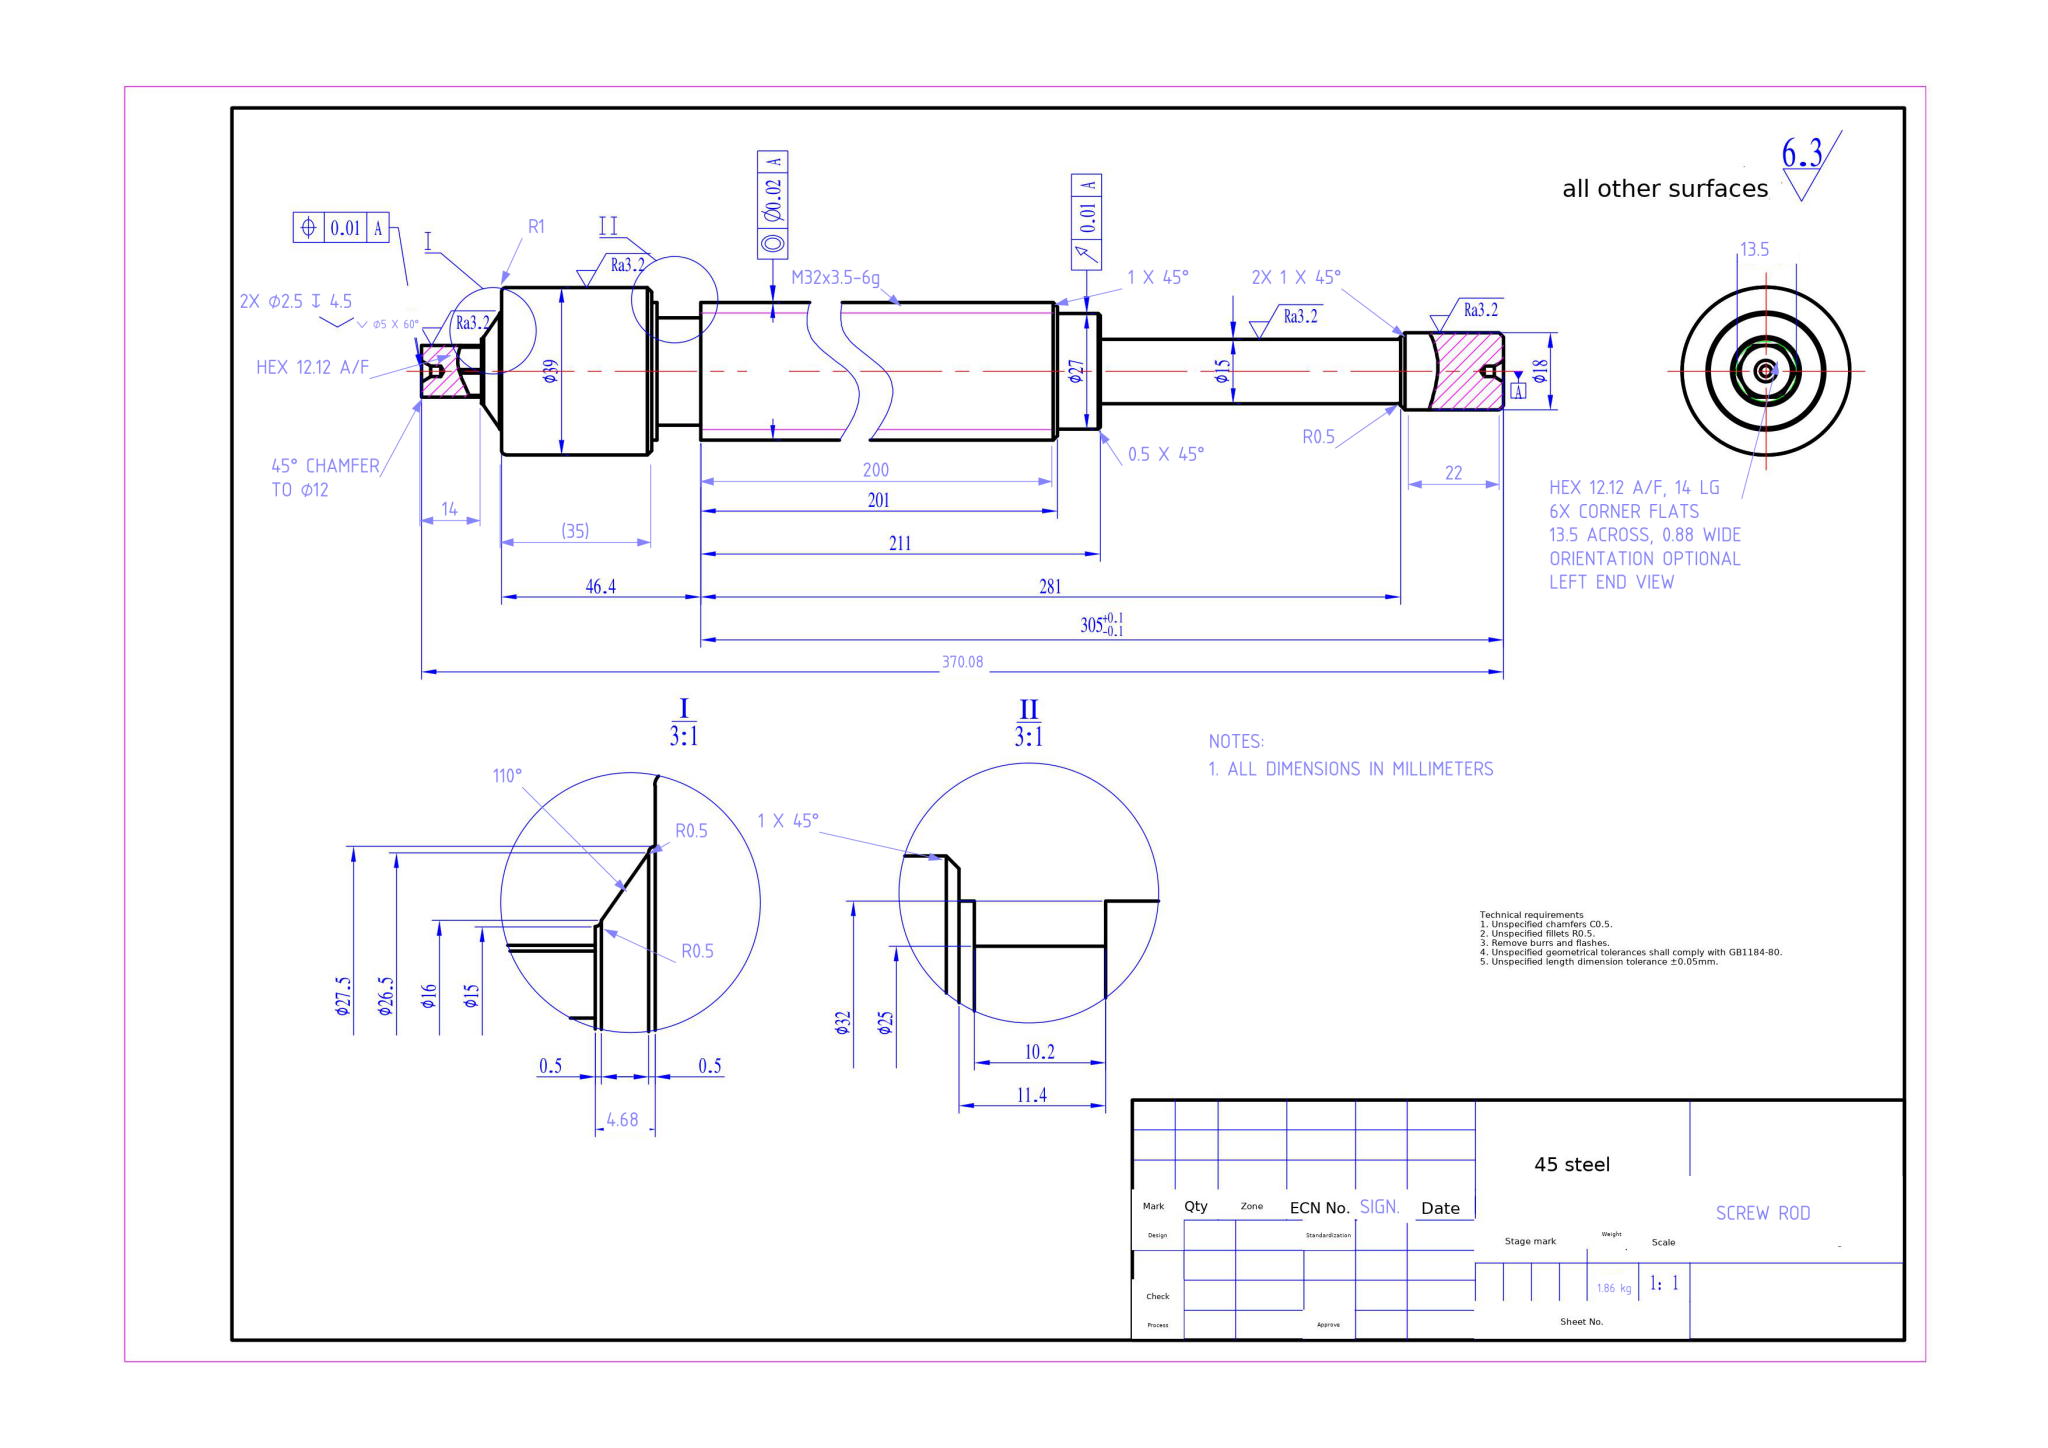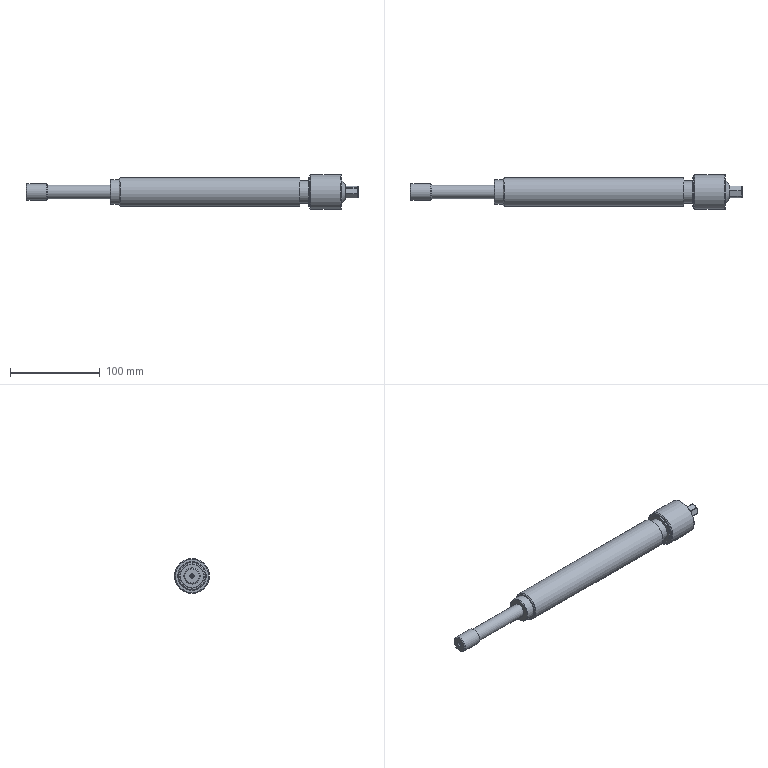Part | NX | mm | 1 solid | 45 faces | box 370.08 x 39 x 39 mm | volume 236852 mm3 | plane 21 | cone 11 | cylinder 9 | torus 4 | commonest cylinder face diameters 32 x2 2.5 x2 18 x1 15 x1 27 x1 25 x1 39 x1